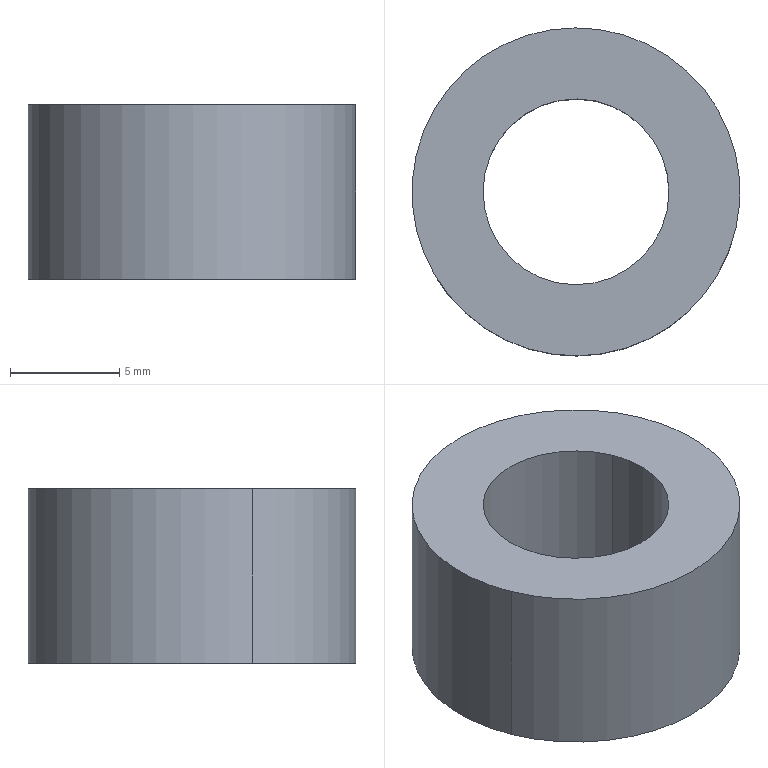Component | SolidWorks | CylinderWasher2-1 | 1 solid | 6 faces | box 15 x 15 x 8 mm | volume 960 mm3 | cylinder 4 | plane 2 | commonest cylinder face diameters 8.5 x2 15 x2
build123d program:
from build123d import *

# Parameters (mm, degrees)
SKETCH1_R           = 7.5
SKETCH1_R_2         = 4.25
BOSS_EXTRUDE1_DEPTH = 8


with BuildPart() as part:
    # Sketch1 → Boss-Extrude1 (new body)
    with BuildSketch(Plane.XY):
        Circle(SKETCH1_R)
        Circle(SKETCH1_R_2, mode=Mode.SUBTRACT)
    extrude(amount=BOSS_EXTRUDE1_DEPTH)


solid = part.part

# Placed as in the assembly
solid = solid.moved(Location((-33.181, 22.568, 7), (0, 0, 0)))
STEP:
#1=COLOUR_RGB('',0.7922,0.8196,0.9333);
#2=FILL_AREA_STYLE_COLOUR('',#1);
#3=FILL_AREA_STYLE('',(#2));
#4=SURFACE_STYLE_FILL_AREA(#3);
#5=SURFACE_SIDE_STYLE('',(#4));
#6=SURFACE_STYLE_USAGE(.BOTH.,#5);
#7=PRESENTATION_STYLE_ASSIGNMENT((#6));
#8=CARTESIAN_POINT('',(-1.151,0.9505,0.5906));
#9=VERTEX_POINT('',#8);
#10=CARTESIAN_POINT('',(-1.462,0.8265,0.5906));
#11=VERTEX_POINT('',#10);
#12=CARTESIAN_POINT('',(-1.306,0.8885,0.5906));
#13=DIRECTION('',(0.,0.,1.));
#14=DIRECTION('',(-0.9287,-0.3707,0.));
#15=AXIS2_PLACEMENT_3D('',#12,#13,#14);
#16=CIRCLE('',#15,0.1673);
#17=EDGE_CURVE('',#9,#11,#16,.T.);
#18=ORIENTED_EDGE('',*,*,#17,.T.);
#19=CARTESIAN_POINT('',(-1.462,0.8265,0.2756));
#20=VERTEX_POINT('',#19);
#21=CARTESIAN_POINT('',(-1.462,0.8265,0.5906));
#22=DIRECTION('',(0.,0.,-1.));
#23=VECTOR('',#22,39.37);
#24=LINE('',#21,#23);
#25=EDGE_CURVE('',#11,#20,#24,.T.);
#26=ORIENTED_EDGE('',*,*,#25,.T.);
#27=CARTESIAN_POINT('',(-1.151,0.9505,0.2756));
#28=VERTEX_POINT('',#27);
#29=CARTESIAN_POINT('',(-1.306,0.8885,0.2756));
#30=DIRECTION('',(0.,0.,1.));
#31=DIRECTION('',(-0.9287,-0.3707,0.));
#32=AXIS2_PLACEMENT_3D('',#29,#30,#31);
#33=CIRCLE('',#32,0.1673);
#34=EDGE_CURVE('',#28,#20,#33,.T.);
#35=ORIENTED_EDGE('',*,*,#34,.F.);
#36=CARTESIAN_POINT('',(-1.151,0.9505,0.5906));
#37=DIRECTION('',(0.,0.,-1.));
#38=VECTOR('',#37,39.37);
#39=LINE('',#36,#38);
#40=EDGE_CURVE('',#9,#28,#39,.T.);
#41=ORIENTED_EDGE('',*,*,#40,.F.);
#42=EDGE_LOOP('',(#18,#26,#35,#41));
#43=FACE_OUTER_BOUND('',#42,.T.);
#44=CARTESIAN_POINT('',(-1.306,0.8885,0.5906));
#45=DIRECTION('',(0.,0.,-1.));
#46=DIRECTION('',(0.9287,0.3707,0.));
#47=AXIS2_PLACEMENT_3D('',#44,#45,#46);
#48=CYLINDRICAL_SURFACE('',#47,0.1673);
#49=ADVANCED_FACE('',(#43),#48,.F.);
#50=CARTESIAN_POINT('',(-1.581,0.779,0.5906));
#51=VERTEX_POINT('',#50);
#52=CARTESIAN_POINT('',(-1.032,0.998,0.5906));
#53=VERTEX_POINT('',#52);
#54=CARTESIAN_POINT('',(-1.306,0.8885,0.5906));
#55=DIRECTION('',(0.,0.,1.));
#56=DIRECTION('',(-0.9287,-0.3707,0.));
#57=AXIS2_PLACEMENT_3D('',#54,#55,#56);
#58=CIRCLE('',#57,0.2953);
#59=EDGE_CURVE('',#51,#53,#58,.T.);
#60=ORIENTED_EDGE('',*,*,#59,.F.);
#61=CARTESIAN_POINT('',(-1.581,0.779,0.2756));
#62=VERTEX_POINT('',#61);
#63=CARTESIAN_POINT('',(-1.581,0.779,0.5906));
#64=DIRECTION('',(0.,0.,-1.));
#65=VECTOR('',#64,39.37);
#66=LINE('',#63,#65);
#67=EDGE_CURVE('',#51,#62,#66,.T.);
#68=ORIENTED_EDGE('',*,*,#67,.T.);
#69=CARTESIAN_POINT('',(-1.032,0.998,0.2756));
#70=VERTEX_POINT('',#69);
#71=CARTESIAN_POINT('',(-1.306,0.8885,0.2756));
#72=DIRECTION('',(0.,0.,1.));
#73=DIRECTION('',(-0.9287,-0.3707,0.));
#74=AXIS2_PLACEMENT_3D('',#71,#72,#73);
#75=CIRCLE('',#74,0.2953);
#76=EDGE_CURVE('',#62,#70,#75,.T.);
#77=ORIENTED_EDGE('',*,*,#76,.T.);
#78=CARTESIAN_POINT('',(-1.032,0.998,0.5906));
#79=DIRECTION('',(0.,0.,-1.));
#80=VECTOR('',#79,39.37);
#81=LINE('',#78,#80);
#82=EDGE_CURVE('',#53,#70,#81,.T.);
#83=ORIENTED_EDGE('',*,*,#82,.F.);
#84=EDGE_LOOP('',(#60,#68,#77,#83));
#85=FACE_OUTER_BOUND('',#84,.T.);
#86=CARTESIAN_POINT('',(-1.306,0.8885,0.5906));
#87=DIRECTION('',(0.,0.,-1.));
#88=DIRECTION('',(0.9287,0.3707,0.));
#89=AXIS2_PLACEMENT_3D('',#86,#87,#88);
#90=CYLINDRICAL_SURFACE('',#89,0.2953);
#91=ADVANCED_FACE('',(#85),#90,.T.);
#92=CARTESIAN_POINT('',(-1.306,0.8885,0.5906));
#93=DIRECTION('',(0.,0.,1.));
#94=DIRECTION('',(-0.9287,-0.3707,0.));
#95=AXIS2_PLACEMENT_3D('',#92,#93,#94);
#96=CIRCLE('',#95,0.2953);
#97=EDGE_CURVE('',#53,#51,#96,.T.);
#98=ORIENTED_EDGE('',*,*,#97,.T.);
#99=ORIENTED_EDGE('',*,*,#59,.T.);
#100=EDGE_LOOP('',(#98,#99));
#101=FACE_OUTER_BOUND('',#100,.T.);
#102=ORIENTED_EDGE('',*,*,#17,.F.);
#103=CARTESIAN_POINT('',(-1.306,0.8885,0.5906));
#104=DIRECTION('',(0.,0.,1.));
#105=DIRECTION('',(-0.9287,-0.3707,0.));
#106=AXIS2_PLACEMENT_3D('',#103,#104,#105);
#107=CIRCLE('',#106,0.1673);
#108=EDGE_CURVE('',#11,#9,#107,.T.);
#109=ORIENTED_EDGE('',*,*,#108,.F.);
#110=EDGE_LOOP('',(#102,#109));
#111=FACE_BOUND('',#110,.T.);
#112=CARTESIAN_POINT('',(-1.306,0.8885,0.5906));
#113=DIRECTION('',(0.,0.,1.));
#114=DIRECTION('',(-0.9287,-0.3707,0.));
#115=AXIS2_PLACEMENT_3D('',#112,#113,#114);
#116=PLANE('',#115);
#117=ADVANCED_FACE('',(#101,#111),#116,.T.);
#118=CARTESIAN_POINT('',(-1.306,0.8885,0.2756));
#119=DIRECTION('',(0.,0.,1.));
#120=DIRECTION('',(-0.9287,-0.3707,0.));
#121=AXIS2_PLACEMENT_3D('',#118,#119,#120);
#122=CIRCLE('',#121,0.2953);
#123=EDGE_CURVE('',#70,#62,#122,.T.);
#124=ORIENTED_EDGE('',*,*,#123,.F.);
#125=ORIENTED_EDGE('',*,*,#76,.F.);
#126=EDGE_LOOP('',(#124,#125));
#127=FACE_OUTER_BOUND('',#126,.T.);
#128=ORIENTED_EDGE('',*,*,#34,.T.);
#129=CARTESIAN_POINT('',(-1.306,0.8885,0.2756));
#130=DIRECTION('',(0.,0.,1.));
#131=DIRECTION('',(-0.9287,-0.3707,0.));
#132=AXIS2_PLACEMENT_3D('',#129,#130,#131);
#133=CIRCLE('',#132,0.1673);
#134=EDGE_CURVE('',#20,#28,#133,.T.);
#135=ORIENTED_EDGE('',*,*,#134,.T.);
#136=EDGE_LOOP('',(#128,#135));
#137=FACE_BOUND('',#136,.T.);
#138=CARTESIAN_POINT('',(-1.306,0.8885,0.2756));
#139=DIRECTION('',(0.,0.,1.));
#140=DIRECTION('',(-0.9287,-0.3707,0.));
#141=AXIS2_PLACEMENT_3D('',#138,#139,#140);
#142=PLANE('',#141);
#143=ADVANCED_FACE('',(#127,#137),#142,.F.);
#144=ORIENTED_EDGE('',*,*,#67,.F.);
#145=ORIENTED_EDGE('',*,*,#97,.F.);
#146=ORIENTED_EDGE('',*,*,#82,.T.);
#147=ORIENTED_EDGE('',*,*,#123,.T.);
#148=EDGE_LOOP('',(#144,#145,#146,#147));
#149=FACE_OUTER_BOUND('',#148,.T.);
#150=CARTESIAN_POINT('',(-1.306,0.8885,0.5906));
#151=DIRECTION('',(0.,0.,-1.));
#152=DIRECTION('',(0.9287,0.3707,0.));
#153=AXIS2_PLACEMENT_3D('',#150,#151,#152);
#154=CYLINDRICAL_SURFACE('',#153,0.2953);
#155=ADVANCED_FACE('',(#149),#154,.T.);
#156=ORIENTED_EDGE('',*,*,#25,.F.);
#157=ORIENTED_EDGE('',*,*,#108,.T.);
#158=ORIENTED_EDGE('',*,*,#40,.T.);
#159=ORIENTED_EDGE('',*,*,#134,.F.);
#160=EDGE_LOOP('',(#156,#157,#158,#159));
#161=FACE_OUTER_BOUND('',#160,.T.);
#162=CARTESIAN_POINT('',(-1.306,0.8885,0.5906));
#163=DIRECTION('',(0.,0.,-1.));
#164=DIRECTION('',(0.9287,0.3707,0.));
#165=AXIS2_PLACEMENT_3D('',#162,#163,#164);
#166=CYLINDRICAL_SURFACE('',#165,0.1673);
#167=ADVANCED_FACE('',(#161),#166,.F.);
#168=CLOSED_SHELL('',(#49,#91,#117,#143,#155,#167));
#169=MANIFOLD_SOLID_BREP('',#168);
#170=STYLED_ITEM('',(#7),#169);
#171=PRESENTATION_LAYER_ASSIGNMENT('','',(#170));
#172=CARTESIAN_POINT('',(0.,0.,0.));
#173=DIRECTION('',(0.,0.,1.));
#174=DIRECTION('',(1.,0.,0.));
#175=AXIS2_PLACEMENT_3D('',#172,#173,#174);
#176=(LENGTH_UNIT()NAMED_UNIT(*)SI_UNIT($,.METRE.));
#177=LENGTH_MEASURE_WITH_UNIT(LENGTH_MEASURE(0.0254),#176);
#178=DIMENSIONAL_EXPONENTS(1.,0.,0.,0.,0.,0.,0.);
#179=(CONVERSION_BASED_UNIT('',#177)LENGTH_UNIT()NAMED_UNIT(#178));
#180=UNCERTAINTY_MEASURE_WITH_UNIT(LENGTH_MEASURE(0.00001),#179,'','');
#181=(NAMED_UNIT(*)PLANE_ANGLE_UNIT()SI_UNIT($,.RADIAN.));
#182=(NAMED_UNIT(*)SI_UNIT($,.STERADIAN.)SOLID_ANGLE_UNIT());
#183=(GEOMETRIC_REPRESENTATION_CONTEXT(3)GLOBAL_UNCERTAINTY_ASSIGNED_CONTEXT((#180))GLOBAL_UNIT_ASSIGNED_CONTEXT((#179,#181,#182))REPRESENTATION_CONTEXT('',''));
#184=ADVANCED_BREP_SHAPE_REPRESENTATION('',(#169,#175),#183);
#185=(LENGTH_UNIT()NAMED_UNIT(*)SI_UNIT($,.METRE.));
#186=LENGTH_MEASURE_WITH_UNIT(LENGTH_MEASURE(0.0254),#185);
#187=DIMENSIONAL_EXPONENTS(1.,0.,0.,0.,0.,0.,0.);
#188=(CONVERSION_BASED_UNIT('',#186)LENGTH_UNIT()NAMED_UNIT(#187));
#189=UNCERTAINTY_MEASURE_WITH_UNIT(LENGTH_MEASURE(0.00001),#188,'','');
#190=(NAMED_UNIT(*)PLANE_ANGLE_UNIT()SI_UNIT($,.RADIAN.));
#191=(NAMED_UNIT(*)SI_UNIT($,.STERADIAN.)SOLID_ANGLE_UNIT());
#192=(GEOMETRIC_REPRESENTATION_CONTEXT(3)GLOBAL_UNCERTAINTY_ASSIGNED_CONTEXT((#189))GLOBAL_UNIT_ASSIGNED_CONTEXT((#188,#190,#191))REPRESENTATION_CONTEXT('',''));
#193=MECHANICAL_DESIGN_GEOMETRIC_PRESENTATION_REPRESENTATION('',(#170),#192);